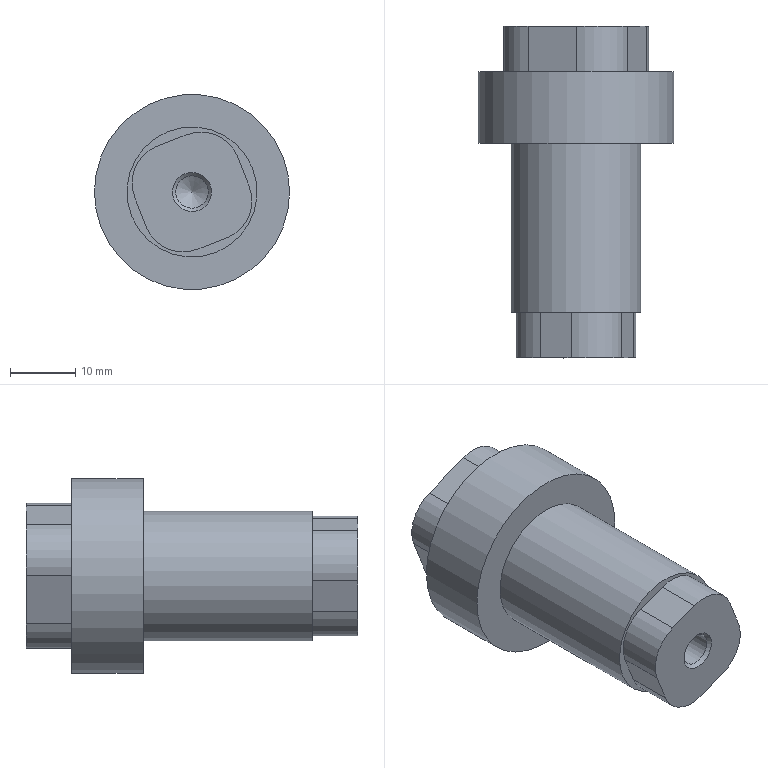Component | NX | ROT_SHAFT | 1 solid | 29 faces | volume 19588 mm3 | plane 13 | cylinder 12 | cone 4 | commonest cylinder face diameters 12 x8 30 x1 20 x1 6.8 x1 5 x1